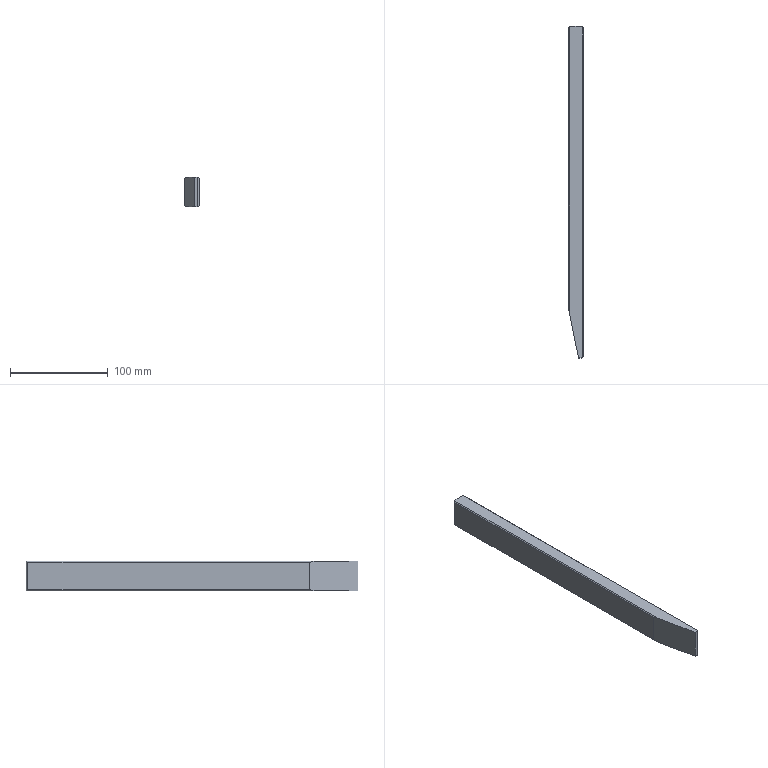Component | SolidWorks | AX00-102.1.1-1_AX00-101.1.1-1_05.1.1-1 | 1 solid | 14 faces | box 15 x 340 x 30 mm | volume 144693 mm3 | plane 14
build123d program:
from build123d import *

# Parameters (mm, degrees)
SKETCH1_W           = 340
SKETCH1_H           = 30
BOSS_EXTRUDE1_DEPTH = 7.5
CHAMFER1_SIZE       = 10
CHAMFER1_SIZE2      = 50
CHAMFER2_SIZE       = 2
CHAMFER3_SIZE       = 1


with BuildPart() as part:
    # Sketch1 → Boss-Extrude1 (new, symmetric)
    with BuildSketch(Plane.XY):
        Rectangle(SKETCH1_W, SKETCH1_H)
    extrude(amount=BOSS_EXTRUDE1_DEPTH, both=True)

    # Chamfer1
    chamfer1_edges = [part.edges().sort_by_distance(p)[0] for p in [
        (170, 0, 7.5),
    ]]
    chamfer1_side = [part.faces().sort_by_distance(p)[0] for p in [
        (170, 0, 0),
    ]]
    chamfer(chamfer1_edges, length=CHAMFER1_SIZE, length2=CHAMFER1_SIZE2, reference=chamfer1_side[0])

    # Chamfer2
    chamfer2_edges = [part.edges().sort_by_distance(p)[0] for p in [
        (-170, 0, 7.5),
        (-170, 0, -7.5),
        (170, 0, -7.5),
    ]]
    chamfer(chamfer2_edges, length=CHAMFER2_SIZE)

    # Chamfer3
    chamfer3_edges = [part.edges().sort_by_distance(p)[0] for p in [
        (-24, 15, 7.5),
        (0, 15, -7.5),
        (0, -15, -7.5),
        (-24, -15, 7.5),
    ]]
    chamfer(chamfer3_edges, length=CHAMFER3_SIZE)


solid = part.part

# Placed as in the assembly
solid = solid.moved(Location((-68.869, 1343.364, 167.5), (90, -90, 0)))